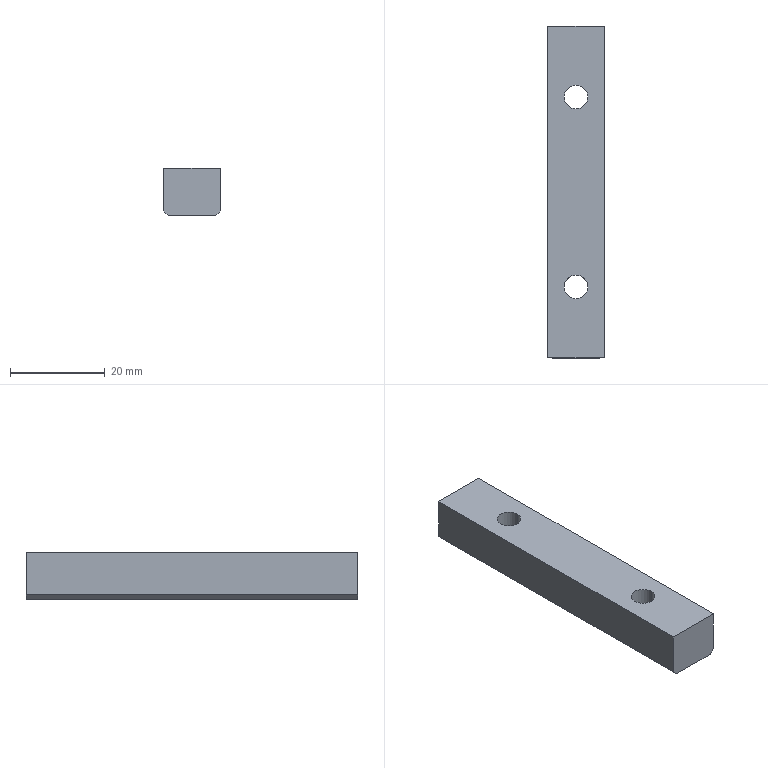Component | SolidWorks | Q1-A12-S21-Q1A.SLDASQ-1_Q1-A12-S21-Q1A-02A-1 | 1 solid | 12 faces | box 12 x 70 x 10 mm | volume 7937 mm3 | plane 8 | cylinder 4 | commonest cylinder face diameters 5 x4 | material Q235-Steel
build123d program:
from build123d import *

# Parameters (mm, degrees)
SKETCH1_W             = 70
SKETCH1_H             = 12
BOSS_EXTRUDE1_DEPTH   = 10
M6X1_0_TAPPED_HOLE1_D = 5
CHAMFER1_SIZE         = 1


with BuildPart() as part:
    # Sketch1 → Boss-Extrude1 (new body)
    with BuildSketch(Plane(origin=(0, 0, 0), x_dir=(1, 0, 0), z_dir=(0, 1, 0))):
        Rectangle(SKETCH1_W, SKETCH1_H)
    extrude(amount=BOSS_EXTRUDE1_DEPTH)

    # M6x1.0 Tapped Hole1 (through all)
    with Locations(Plane(origin=(0, 10, 0), x_dir=(1, 0, 0), z_dir=(0, 1, 0))):
        with Locations((20, 0), (-20, 0)):
            Hole(M6X1_0_TAPPED_HOLE1_D / 2)

    # Chamfer1
    chamfer1_edges = [part.edges().sort_by_distance(p)[0] for p in [
        (0, 10, 6),
        (0, 10, -6),
    ]]
    chamfer(chamfer1_edges, length=CHAMFER1_SIZE)


solid = part.part

# Placed as in the assembly
solid = solid.moved(Location((42.5, 0, -142.5), (-90, 90, 0)))
STEP:
#1=COLOUR_RGB('',0.7922,0.8196,0.9333);
#2=FILL_AREA_STYLE_COLOUR('',#1);
#3=FILL_AREA_STYLE('',(#2));
#4=SURFACE_STYLE_FILL_AREA(#3);
#5=SURFACE_SIDE_STYLE('',(#4));
#6=SURFACE_STYLE_USAGE(.BOTH.,#5);
#7=PRESENTATION_STYLE_ASSIGNMENT((#6));
#8=CARTESIAN_POINT('',(1.575,-0.7874,-5.61));
#9=VERTEX_POINT('',#8);
#10=CARTESIAN_POINT('',(1.772,-0.7874,-5.61));
#11=VERTEX_POINT('',#10);
#12=CARTESIAN_POINT('',(1.673,-0.7874,-5.61));
#13=DIRECTION('',(0.,-0.,-1.));
#14=DIRECTION('',(1.,0.,0.));
#15=AXIS2_PLACEMENT_3D('',#12,#13,#14);
#16=CIRCLE('',#15,0.09843);
#17=EDGE_CURVE('',#9,#11,#16,.T.);
#18=ORIENTED_EDGE('',*,*,#17,.F.);
#19=CARTESIAN_POINT('',(1.575,-0.7874,-6.004));
#20=VERTEX_POINT('',#19);
#21=CARTESIAN_POINT('',(1.575,-0.7874,-6.004));
#22=DIRECTION('',(0.,-0.,-1.));
#23=VECTOR('',#22,39.37);
#24=LINE('',#21,#23);
#25=EDGE_CURVE('',#9,#20,#24,.T.);
#26=ORIENTED_EDGE('',*,*,#25,.T.);
#27=CARTESIAN_POINT('',(1.772,-0.7874,-6.004));
#28=VERTEX_POINT('',#27);
#29=CARTESIAN_POINT('',(1.673,-0.7874,-6.004));
#30=DIRECTION('',(0.,-0.,-1.));
#31=DIRECTION('',(1.,0.,0.));
#32=AXIS2_PLACEMENT_3D('',#29,#30,#31);
#33=CIRCLE('',#32,0.09843);
#34=EDGE_CURVE('',#20,#28,#33,.T.);
#35=ORIENTED_EDGE('',*,*,#34,.T.);
#36=CARTESIAN_POINT('',(1.772,-0.7874,-6.004));
#37=DIRECTION('',(0.,-0.,-1.));
#38=VECTOR('',#37,39.37);
#39=LINE('',#36,#38);
#40=EDGE_CURVE('',#11,#28,#39,.T.);
#41=ORIENTED_EDGE('',*,*,#40,.F.);
#42=EDGE_LOOP('',(#18,#26,#35,#41));
#43=FACE_OUTER_BOUND('',#42,.T.);
#44=CARTESIAN_POINT('',(1.673,-0.7874,-6.004));
#45=DIRECTION('',(0.,-0.,-1.));
#46=DIRECTION('',(1.,0.,0.));
#47=AXIS2_PLACEMENT_3D('',#44,#45,#46);
#48=CYLINDRICAL_SURFACE('',#47,0.09843);
#49=ADVANCED_FACE('',(#43),#48,.F.);
#50=CARTESIAN_POINT('',(1.575,0.7874,-5.61));
#51=VERTEX_POINT('',#50);
#52=CARTESIAN_POINT('',(1.772,0.7874,-5.61));
#53=VERTEX_POINT('',#52);
#54=CARTESIAN_POINT('',(1.673,0.7874,-5.61));
#55=DIRECTION('',(0.,-0.,-1.));
#56=DIRECTION('',(1.,0.,0.));
#57=AXIS2_PLACEMENT_3D('',#54,#55,#56);
#58=CIRCLE('',#57,0.09843);
#59=EDGE_CURVE('',#51,#53,#58,.T.);
#60=ORIENTED_EDGE('',*,*,#59,.F.);
#61=CARTESIAN_POINT('',(1.575,0.7874,-6.004));
#62=VERTEX_POINT('',#61);
#63=CARTESIAN_POINT('',(1.575,0.7874,-6.004));
#64=DIRECTION('',(0.,-0.,-1.));
#65=VECTOR('',#64,39.37);
#66=LINE('',#63,#65);
#67=EDGE_CURVE('',#51,#62,#66,.T.);
#68=ORIENTED_EDGE('',*,*,#67,.T.);
#69=CARTESIAN_POINT('',(1.772,0.7874,-6.004));
#70=VERTEX_POINT('',#69);
#71=CARTESIAN_POINT('',(1.673,0.7874,-6.004));
#72=DIRECTION('',(0.,-0.,-1.));
#73=DIRECTION('',(1.,0.,0.));
#74=AXIS2_PLACEMENT_3D('',#71,#72,#73);
#75=CIRCLE('',#74,0.09843);
#76=EDGE_CURVE('',#62,#70,#75,.T.);
#77=ORIENTED_EDGE('',*,*,#76,.T.);
#78=CARTESIAN_POINT('',(1.772,0.7874,-6.004));
#79=DIRECTION('',(0.,-0.,-1.));
#80=VECTOR('',#79,39.37);
#81=LINE('',#78,#80);
#82=EDGE_CURVE('',#53,#70,#81,.T.);
#83=ORIENTED_EDGE('',*,*,#82,.F.);
#84=EDGE_LOOP('',(#60,#68,#77,#83));
#85=FACE_OUTER_BOUND('',#84,.T.);
#86=CARTESIAN_POINT('',(1.673,0.7874,-6.004));
#87=DIRECTION('',(0.,-0.,-1.));
#88=DIRECTION('',(1.,0.,0.));
#89=AXIS2_PLACEMENT_3D('',#86,#87,#88);
#90=CYLINDRICAL_SURFACE('',#89,0.09843);
#91=ADVANCED_FACE('',(#85),#90,.F.);
#92=CARTESIAN_POINT('',(1.437,-1.378,-5.965));
#93=VERTEX_POINT('',#92);
#94=CARTESIAN_POINT('',(1.437,-1.378,-5.61));
#95=VERTEX_POINT('',#94);
#96=CARTESIAN_POINT('',(1.437,-1.378,-6.004));
#97=DIRECTION('',(-0.,0.,1.));
#98=VECTOR('',#97,39.37);
#99=LINE('',#96,#98);
#100=EDGE_CURVE('',#93,#95,#99,.T.);
#101=ORIENTED_EDGE('',*,*,#100,.F.);
#102=CARTESIAN_POINT('',(1.476,-1.378,-6.004));
#103=VERTEX_POINT('',#102);
#104=CARTESIAN_POINT('',(1.476,-1.378,-6.004));
#105=DIRECTION('',(0.7071,0.,-0.7071));
#106=VECTOR('',#105,39.37);
#107=LINE('',#104,#106);
#108=EDGE_CURVE('',#93,#103,#107,.T.);
#109=ORIENTED_EDGE('',*,*,#108,.T.);
#110=CARTESIAN_POINT('',(1.87,-1.378,-6.004));
#111=VERTEX_POINT('',#110);
#112=CARTESIAN_POINT('',(1.909,-1.378,-6.004));
#113=DIRECTION('',(-1.,-0.,-0.));
#114=VECTOR('',#113,39.37);
#115=LINE('',#112,#114);
#116=EDGE_CURVE('',#111,#103,#115,.T.);
#117=ORIENTED_EDGE('',*,*,#116,.F.);
#118=CARTESIAN_POINT('',(1.909,-1.378,-5.965));
#119=VERTEX_POINT('',#118);
#120=CARTESIAN_POINT('',(1.87,-1.378,-6.004));
#121=DIRECTION('',(0.7071,0.,0.7071));
#122=VECTOR('',#121,39.37);
#123=LINE('',#120,#122);
#124=EDGE_CURVE('',#111,#119,#123,.T.);
#125=ORIENTED_EDGE('',*,*,#124,.T.);
#126=CARTESIAN_POINT('',(1.909,-1.378,-5.61));
#127=VERTEX_POINT('',#126);
#128=CARTESIAN_POINT('',(1.909,-1.378,-6.004));
#129=DIRECTION('',(-0.,0.,1.));
#130=VECTOR('',#129,39.37);
#131=LINE('',#128,#130);
#132=EDGE_CURVE('',#119,#127,#131,.T.);
#133=ORIENTED_EDGE('',*,*,#132,.T.);
#134=CARTESIAN_POINT('',(1.909,-1.378,-5.61));
#135=DIRECTION('',(-1.,-0.,-0.));
#136=VECTOR('',#135,39.37);
#137=LINE('',#134,#136);
#138=EDGE_CURVE('',#127,#95,#137,.T.);
#139=ORIENTED_EDGE('',*,*,#138,.T.);
#140=EDGE_LOOP('',(#101,#109,#117,#125,#133,#139));
#141=FACE_OUTER_BOUND('',#140,.T.);
#142=CARTESIAN_POINT('',(1.909,-1.378,-6.004));
#143=DIRECTION('',(-0.,1.,-0.));
#144=DIRECTION('',(1.,0.,0.));
#145=AXIS2_PLACEMENT_3D('',#142,#143,#144);
#146=PLANE('',#145);
#147=ADVANCED_FACE('',(#141),#146,.F.);
#148=CARTESIAN_POINT('',(1.437,1.378,-5.965));
#149=VERTEX_POINT('',#148);
#150=CARTESIAN_POINT('',(1.437,1.378,-5.61));
#151=VERTEX_POINT('',#150);
#152=CARTESIAN_POINT('',(1.437,1.378,-6.004));
#153=DIRECTION('',(-0.,0.,1.));
#154=VECTOR('',#153,39.37);
#155=LINE('',#152,#154);
#156=EDGE_CURVE('',#149,#151,#155,.T.);
#157=ORIENTED_EDGE('',*,*,#156,.F.);
#158=CARTESIAN_POINT('',(1.437,1.378,-5.965));
#159=DIRECTION('',(0.,-1.,0.));
#160=VECTOR('',#159,39.37);
#161=LINE('',#158,#160);
#162=EDGE_CURVE('',#149,#93,#161,.T.);
#163=ORIENTED_EDGE('',*,*,#162,.T.);
#164=ORIENTED_EDGE('',*,*,#100,.T.);
#165=CARTESIAN_POINT('',(1.437,1.378,-5.61));
#166=DIRECTION('',(-0.,1.,-0.));
#167=VECTOR('',#166,39.37);
#168=LINE('',#165,#167);
#169=EDGE_CURVE('',#95,#151,#168,.T.);
#170=ORIENTED_EDGE('',*,*,#169,.T.);
#171=EDGE_LOOP('',(#157,#163,#164,#170));
#172=FACE_OUTER_BOUND('',#171,.T.);
#173=CARTESIAN_POINT('',(1.437,1.378,-6.004));
#174=DIRECTION('',(1.,0.,0.));
#175=DIRECTION('',(0.,-1.,0.));
#176=AXIS2_PLACEMENT_3D('',#173,#174,#175);
#177=PLANE('',#176);
#178=ADVANCED_FACE('',(#172),#177,.F.);
#179=CARTESIAN_POINT('',(1.476,1.378,-6.004));
#180=VERTEX_POINT('',#179);
#181=CARTESIAN_POINT('',(1.87,1.378,-6.004));
#182=VERTEX_POINT('',#181);
#183=CARTESIAN_POINT('',(1.909,1.378,-6.004));
#184=DIRECTION('',(1.,0.,0.));
#185=VECTOR('',#184,39.37);
#186=LINE('',#183,#185);
#187=EDGE_CURVE('',#180,#182,#186,.T.);
#188=ORIENTED_EDGE('',*,*,#187,.F.);
#189=CARTESIAN_POINT('',(1.476,1.378,-6.004));
#190=DIRECTION('',(-0.7071,-0.,0.7071));
#191=VECTOR('',#190,39.37);
#192=LINE('',#189,#191);
#193=EDGE_CURVE('',#180,#149,#192,.T.);
#194=ORIENTED_EDGE('',*,*,#193,.T.);
#195=ORIENTED_EDGE('',*,*,#156,.T.);
#196=CARTESIAN_POINT('',(1.909,1.378,-5.61));
#197=VERTEX_POINT('',#196);
#198=CARTESIAN_POINT('',(1.909,1.378,-5.61));
#199=DIRECTION('',(1.,0.,0.));
#200=VECTOR('',#199,39.37);
#201=LINE('',#198,#200);
#202=EDGE_CURVE('',#151,#197,#201,.T.);
#203=ORIENTED_EDGE('',*,*,#202,.T.);
#204=CARTESIAN_POINT('',(1.909,1.378,-5.965));
#205=VERTEX_POINT('',#204);
#206=CARTESIAN_POINT('',(1.909,1.378,-6.004));
#207=DIRECTION('',(-0.,0.,1.));
#208=VECTOR('',#207,39.37);
#209=LINE('',#206,#208);
#210=EDGE_CURVE('',#205,#197,#209,.T.);
#211=ORIENTED_EDGE('',*,*,#210,.F.);
#212=CARTESIAN_POINT('',(1.87,1.378,-6.004));
#213=DIRECTION('',(-0.7071,-0.,-0.7071));
#214=VECTOR('',#213,39.37);
#215=LINE('',#212,#214);
#216=EDGE_CURVE('',#205,#182,#215,.T.);
#217=ORIENTED_EDGE('',*,*,#216,.T.);
#218=EDGE_LOOP('',(#188,#194,#195,#203,#211,#217));
#219=FACE_OUTER_BOUND('',#218,.T.);
#220=CARTESIAN_POINT('',(1.909,1.378,-6.004));
#221=DIRECTION('',(0.,-1.,0.));
#222=DIRECTION('',(-1.,-0.,-0.));
#223=AXIS2_PLACEMENT_3D('',#220,#221,#222);
#224=PLANE('',#223);
#225=ADVANCED_FACE('',(#219),#224,.F.);
#226=ORIENTED_EDGE('',*,*,#132,.F.);
#227=CARTESIAN_POINT('',(1.909,1.378,-5.965));
#228=DIRECTION('',(-0.,1.,-0.));
#229=VECTOR('',#228,39.37);
#230=LINE('',#227,#229);
#231=EDGE_CURVE('',#119,#205,#230,.T.);
#232=ORIENTED_EDGE('',*,*,#231,.T.);
#233=ORIENTED_EDGE('',*,*,#210,.T.);
#234=CARTESIAN_POINT('',(1.909,1.378,-5.61));
#235=DIRECTION('',(0.,-1.,0.));
#236=VECTOR('',#235,39.37);
#237=LINE('',#234,#236);
#238=EDGE_CURVE('',#197,#127,#237,.T.);
#239=ORIENTED_EDGE('',*,*,#238,.T.);
#240=EDGE_LOOP('',(#226,#232,#233,#239));
#241=FACE_OUTER_BOUND('',#240,.T.);
#242=CARTESIAN_POINT('',(1.909,1.378,-6.004));
#243=DIRECTION('',(-1.,-0.,-0.));
#244=DIRECTION('',(-0.,1.,-0.));
#245=AXIS2_PLACEMENT_3D('',#242,#243,#244);
#246=PLANE('',#245);
#247=ADVANCED_FACE('',(#241),#246,.F.);
#248=CARTESIAN_POINT('',(1.673,-0.7874,-6.004));
#249=DIRECTION('',(0.,-0.,-1.));
#250=DIRECTION('',(1.,0.,0.));
#251=AXIS2_PLACEMENT_3D('',#248,#249,#250);
#252=CIRCLE('',#251,0.09843);
#253=EDGE_CURVE('',#28,#20,#252,.T.);
#254=ORIENTED_EDGE('',*,*,#253,.F.);
#255=ORIENTED_EDGE('',*,*,#34,.F.);
#256=EDGE_LOOP('',(#254,#255));
#257=FACE_BOUND('',#256,.T.);
#258=CARTESIAN_POINT('',(1.673,0.7874,-6.004));
#259=DIRECTION('',(0.,-0.,-1.));
#260=DIRECTION('',(1.,0.,0.));
#261=AXIS2_PLACEMENT_3D('',#258,#259,#260);
#262=CIRCLE('',#261,0.09843);
#263=EDGE_CURVE('',#70,#62,#262,.T.);
#264=ORIENTED_EDGE('',*,*,#263,.F.);
#265=ORIENTED_EDGE('',*,*,#76,.F.);
#266=EDGE_LOOP('',(#264,#265));
#267=FACE_BOUND('',#266,.T.);
#268=ORIENTED_EDGE('',*,*,#116,.T.);
#269=CARTESIAN_POINT('',(1.476,-0.,-6.004));
#270=DIRECTION('',(-0.,1.,-0.));
#271=VECTOR('',#270,39.37);
#272=LINE('',#269,#271);
#273=EDGE_CURVE('',#103,#180,#272,.T.);
#274=ORIENTED_EDGE('',*,*,#273,.T.);
#275=ORIENTED_EDGE('',*,*,#187,.T.);
#276=CARTESIAN_POINT('',(1.87,0.,-6.004));
#277=DIRECTION('',(0.,-1.,0.));
#278=VECTOR('',#277,39.37);
#279=LINE('',#276,#278);
#280=EDGE_CURVE('',#182,#111,#279,.T.);
#281=ORIENTED_EDGE('',*,*,#280,.T.);
#282=EDGE_LOOP('',(#268,#274,#275,#281));
#283=FACE_OUTER_BOUND('',#282,.T.);
#284=CARTESIAN_POINT('',(1.673,-0.,-6.004));
#285=DIRECTION('',(-0.,0.,1.));
#286=DIRECTION('',(-1.,-0.,-0.));
#287=AXIS2_PLACEMENT_3D('',#284,#285,#286);
#288=PLANE('',#287);
#289=ADVANCED_FACE('',(#257,#267,#283),#288,.F.);
#290=CARTESIAN_POINT('',(1.673,-0.7874,-5.61));
#291=DIRECTION('',(0.,-0.,-1.));
#292=DIRECTION('',(1.,0.,0.));
#293=AXIS2_PLACEMENT_3D('',#290,#291,#292);
#294=CIRCLE('',#293,0.09843);
#295=EDGE_CURVE('',#11,#9,#294,.T.);
#296=ORIENTED_EDGE('',*,*,#295,.T.);
#297=ORIENTED_EDGE('',*,*,#17,.T.);
#298=EDGE_LOOP('',(#296,#297));
#299=FACE_BOUND('',#298,.T.);
#300=CARTESIAN_POINT('',(1.673,0.7874,-5.61));
#301=DIRECTION('',(0.,-0.,-1.));
#302=DIRECTION('',(1.,0.,0.));
#303=AXIS2_PLACEMENT_3D('',#300,#301,#302);
#304=CIRCLE('',#303,0.09843);
#305=EDGE_CURVE('',#53,#51,#304,.T.);
#306=ORIENTED_EDGE('',*,*,#305,.T.);
#307=ORIENTED_EDGE('',*,*,#59,.T.);
#308=EDGE_LOOP('',(#306,#307));
#309=FACE_BOUND('',#308,.T.);
#310=ORIENTED_EDGE('',*,*,#138,.F.);
#311=ORIENTED_EDGE('',*,*,#238,.F.);
#312=ORIENTED_EDGE('',*,*,#202,.F.);
#313=ORIENTED_EDGE('',*,*,#169,.F.);
#314=EDGE_LOOP('',(#310,#311,#312,#313));
#315=FACE_OUTER_BOUND('',#314,.T.);
#316=CARTESIAN_POINT('',(1.673,-0.,-5.61));
#317=DIRECTION('',(-0.,0.,1.));
#318=DIRECTION('',(-1.,-0.,-0.));
#319=AXIS2_PLACEMENT_3D('',#316,#317,#318);
#320=PLANE('',#319);
#321=ADVANCED_FACE('',(#299,#309,#315),#320,.T.);
#322=ORIENTED_EDGE('',*,*,#67,.F.);
#323=ORIENTED_EDGE('',*,*,#305,.F.);
#324=ORIENTED_EDGE('',*,*,#82,.T.);
#325=ORIENTED_EDGE('',*,*,#263,.T.);
#326=EDGE_LOOP('',(#322,#323,#324,#325));
#327=FACE_OUTER_BOUND('',#326,.T.);
#328=CARTESIAN_POINT('',(1.673,0.7874,-6.004));
#329=DIRECTION('',(0.,-0.,-1.));
#330=DIRECTION('',(1.,0.,0.));
#331=AXIS2_PLACEMENT_3D('',#328,#329,#330);
#332=CYLINDRICAL_SURFACE('',#331,0.09843);
#333=ADVANCED_FACE('',(#327),#332,.F.);
#334=ORIENTED_EDGE('',*,*,#25,.F.);
#335=ORIENTED_EDGE('',*,*,#295,.F.);
#336=ORIENTED_EDGE('',*,*,#40,.T.);
#337=ORIENTED_EDGE('',*,*,#253,.T.);
#338=EDGE_LOOP('',(#334,#335,#336,#337));
#339=FACE_OUTER_BOUND('',#338,.T.);
#340=CARTESIAN_POINT('',(1.673,-0.7874,-6.004));
#341=DIRECTION('',(0.,-0.,-1.));
#342=DIRECTION('',(1.,0.,0.));
#343=AXIS2_PLACEMENT_3D('',#340,#341,#342);
#344=CYLINDRICAL_SURFACE('',#343,0.09843);
#345=ADVANCED_FACE('',(#339),#344,.F.);
#346=ORIENTED_EDGE('',*,*,#108,.F.);
#347=ORIENTED_EDGE('',*,*,#162,.F.);
#348=ORIENTED_EDGE('',*,*,#193,.F.);
#349=ORIENTED_EDGE('',*,*,#273,.F.);
#350=EDGE_LOOP('',(#346,#347,#348,#349));
#351=FACE_OUTER_BOUND('',#350,.T.);
#352=CARTESIAN_POINT('',(1.476,-0.,-6.004));
#353=DIRECTION('',(0.7071,0.,0.7071));
#354=DIRECTION('',(-0.,1.,-0.));
#355=AXIS2_PLACEMENT_3D('',#352,#353,#354);
#356=PLANE('',#355);
#357=ADVANCED_FACE('',(#351),#356,.F.);
#358=ORIENTED_EDGE('',*,*,#216,.F.);
#359=ORIENTED_EDGE('',*,*,#231,.F.);
#360=ORIENTED_EDGE('',*,*,#124,.F.);
#361=ORIENTED_EDGE('',*,*,#280,.F.);
#362=EDGE_LOOP('',(#358,#359,#360,#361));
#363=FACE_OUTER_BOUND('',#362,.T.);
#364=CARTESIAN_POINT('',(1.87,0.,-6.004));
#365=DIRECTION('',(-0.7071,-0.,0.7071));
#366=DIRECTION('',(0.,-1.,0.));
#367=AXIS2_PLACEMENT_3D('',#364,#365,#366);
#368=PLANE('',#367);
#369=ADVANCED_FACE('',(#363),#368,.F.);
#370=CLOSED_SHELL('',(#49,#91,#147,#178,#225,#247,#289,#321,#333,#345,#357,#369));
#371=MANIFOLD_SOLID_BREP('',#370);
#372=STYLED_ITEM('',(#7),#371);
#373=PRESENTATION_LAYER_ASSIGNMENT('','',(#372));
#374=(LENGTH_UNIT()NAMED_UNIT(*)SI_UNIT($,.METRE.));
#375=LENGTH_MEASURE_WITH_UNIT(LENGTH_MEASURE(0.0254),#374);
#376=DIMENSIONAL_EXPONENTS(1.,0.,0.,0.,0.,0.,0.);
#377=(CONVERSION_BASED_UNIT('',#375)LENGTH_UNIT()NAMED_UNIT(#376));
#378=UNCERTAINTY_MEASURE_WITH_UNIT(LENGTH_MEASURE(0.00001),#377,'','');
#379=(NAMED_UNIT(*)PLANE_ANGLE_UNIT()SI_UNIT($,.RADIAN.));
#380=(NAMED_UNIT(*)SI_UNIT($,.STERADIAN.)SOLID_ANGLE_UNIT());
#381=(GEOMETRIC_REPRESENTATION_CONTEXT(3)GLOBAL_UNCERTAINTY_ASSIGNED_CONTEXT((#378))GLOBAL_UNIT_ASSIGNED_CONTEXT((#377,#379,#380))REPRESENTATION_CONTEXT('',''));
#382=MECHANICAL_DESIGN_GEOMETRIC_PRESENTATION_REPRESENTATION('',(#372),#381);
#383=CARTESIAN_POINT('',(0.,0.,0.));
#384=DIRECTION('',(0.,0.,1.));
#385=DIRECTION('',(1.,0.,0.));
#386=AXIS2_PLACEMENT_3D('',#383,#384,#385);
#387=(LENGTH_UNIT()NAMED_UNIT(*)SI_UNIT($,.METRE.));
#388=LENGTH_MEASURE_WITH_UNIT(LENGTH_MEASURE(0.0254),#387);
#389=DIMENSIONAL_EXPONENTS(1.,0.,0.,0.,0.,0.,0.);
#390=(CONVERSION_BASED_UNIT('',#388)LENGTH_UNIT()NAMED_UNIT(#389));
#391=UNCERTAINTY_MEASURE_WITH_UNIT(LENGTH_MEASURE(0.00001),#390,'','');
#392=(NAMED_UNIT(*)PLANE_ANGLE_UNIT()SI_UNIT($,.RADIAN.));
#393=(NAMED_UNIT(*)SI_UNIT($,.STERADIAN.)SOLID_ANGLE_UNIT());
#394=(GEOMETRIC_REPRESENTATION_CONTEXT(3)GLOBAL_UNCERTAINTY_ASSIGNED_CONTEXT((#391))GLOBAL_UNIT_ASSIGNED_CONTEXT((#390,#392,#393))REPRESENTATION_CONTEXT('',''));
#395=ADVANCED_BREP_SHAPE_REPRESENTATION('',(#371,#386),#394);